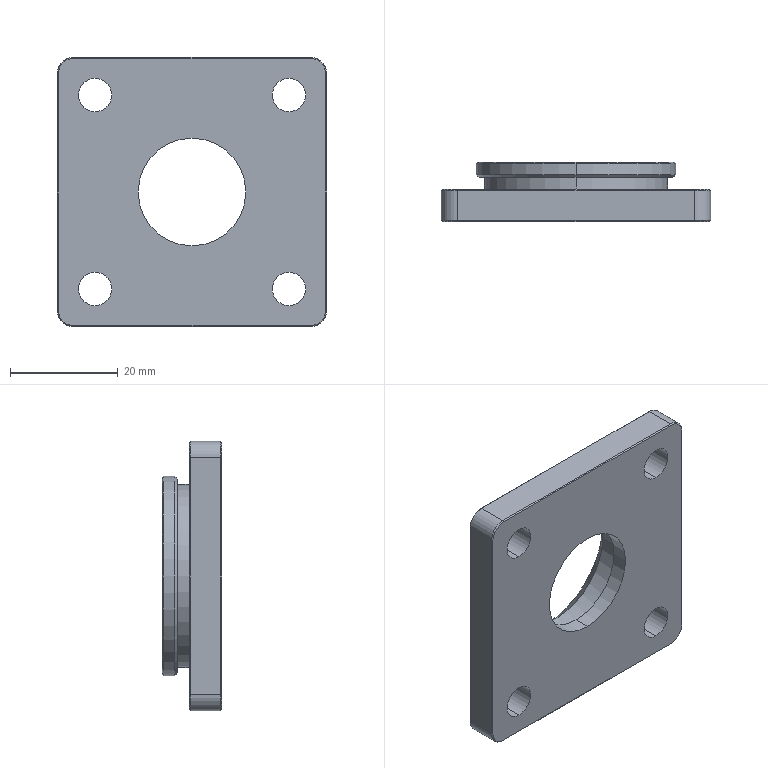CAM job | Mastercam | mm | 4 operations | part box 50 x 11 x 50
1. Contour (Ramp) | 9 - 10 平铣刀
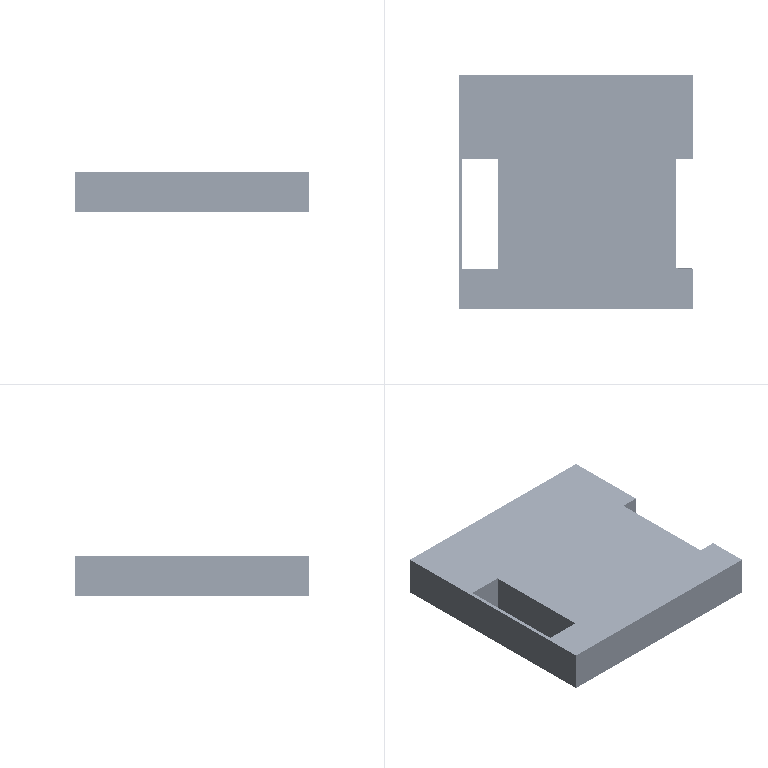2. Contour (2D) | 9 - 10 平铣刀
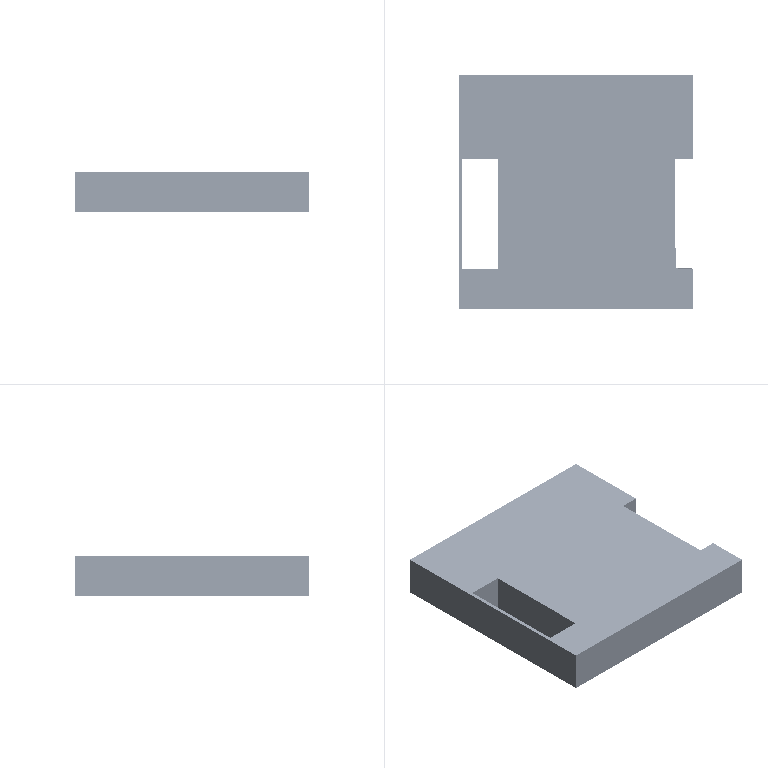3. Drill/Counterbore | 5 - 4 倒角刀
4. Contour (2D chamfer) | 5 - 4 倒角刀